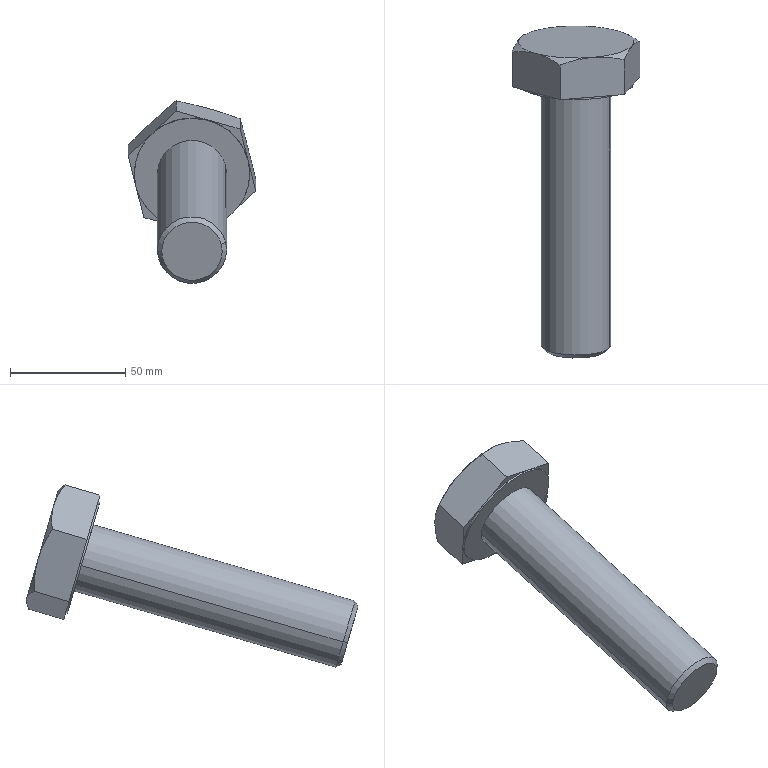Component | SolidWorks | hex structural bolt gradec short_iso-10 | 1 solid | 27 faces | box 55.43 x 143.81 x 78.96 mm | volume 124846 mm3 | plane 15 | cone 8 | cylinder 4 | commonest cylinder face diameters 50 x2 30 x2
STEP:
#1=CARTESIAN_POINT('',(-29.949,-0.9466,13.504));
#2=VERTEX_POINT('',#1);
#3=CARTESIAN_POINT('',(-31.862,-0.8156,13.055));
#4=VERTEX_POINT('',#3);
#5=CARTESIAN_POINT('',(-30.906,-0.8811,13.28));
#6=DIRECTION('',(0.,-0.9601,-0.2797));
#7=DIRECTION('',(0.9713,-0.06652,0.2283));
#8=AXIS2_PLACEMENT_3D('',#5,#6,#7);
#9=CIRCLE('',#8,0.9843);
#10=EDGE_CURVE('',#2,#4,#9,.T.);
#11=ORIENTED_EDGE('',*,*,#10,.F.);
#12=CARTESIAN_POINT('',(-29.949,-0.9163,13.513));
#13=VERTEX_POINT('',#12);
#14=CARTESIAN_POINT('',(-29.949,-0.2397,13.71));
#15=DIRECTION('',(-0.,0.9601,0.2797));
#16=VECTOR('',#15,39.37);
#17=LINE('',#14,#16);
#18=EDGE_CURVE('',#2,#13,#17,.T.);
#19=ORIENTED_EDGE('',*,*,#18,.T.);
#20=CARTESIAN_POINT('',(-30.63,-1.115,14.196));
#21=VERTEX_POINT('',#20);
#22=CARTESIAN_POINT('',(-30.906,-0.8509,13.289));
#23=DIRECTION('',(-0.,0.9601,0.2797));
#24=DIRECTION('',(-0.9713,0.06652,-0.2283));
#25=AXIS2_PLACEMENT_3D('',#22,#23,#24);
#26=CIRCLE('',#25,0.9843);
#27=EDGE_CURVE('',#21,#13,#26,.T.);
#28=ORIENTED_EDGE('',*,*,#27,.F.);
#29=CARTESIAN_POINT('',(-31.586,-1.05,13.971));
#30=VERTEX_POINT('',#29);
#31=CARTESIAN_POINT('',(-30.906,-0.8509,13.289));
#32=DIRECTION('',(-0.,0.9601,0.2797));
#33=DIRECTION('',(-0.9713,0.06652,-0.2283));
#34=AXIS2_PLACEMENT_3D('',#31,#32,#33);
#35=CIRCLE('',#34,0.9843);
#36=EDGE_CURVE('',#30,#21,#35,.T.);
#37=ORIENTED_EDGE('',*,*,#36,.F.);
#38=CARTESIAN_POINT('',(-31.862,-0.7854,13.064));
#39=VERTEX_POINT('',#38);
#40=CARTESIAN_POINT('',(-30.906,-0.8509,13.289));
#41=DIRECTION('',(-0.,0.9601,0.2797));
#42=DIRECTION('',(-0.9713,0.06652,-0.2283));
#43=AXIS2_PLACEMENT_3D('',#40,#41,#42);
#44=CIRCLE('',#43,0.9843);
#45=EDGE_CURVE('',#39,#30,#44,.T.);
#46=ORIENTED_EDGE('',*,*,#45,.F.);
#47=CARTESIAN_POINT('',(-31.862,-0.1088,13.261));
#48=DIRECTION('',(-0.,0.9601,0.2797));
#49=VECTOR('',#48,39.37);
#50=LINE('',#47,#49);
#51=EDGE_CURVE('',#4,#39,#50,.T.);
#52=ORIENTED_EDGE('',*,*,#51,.F.);
#53=EDGE_LOOP('',(#11,#19,#28,#37,#46,#52));
#54=FACE_OUTER_BOUND('',#53,.T.);
#55=CARTESIAN_POINT('',(-30.906,-0.1743,13.486));
#56=DIRECTION('',(-0.,0.9601,0.2797));
#57=DIRECTION('',(-0.9713,0.06652,-0.2283));
#58=AXIS2_PLACEMENT_3D('',#55,#56,#57);
#59=CYLINDRICAL_SURFACE('',#58,0.9843);
#60=ADVANCED_FACE('',(#54),#59,.T.);
#61=CARTESIAN_POINT('',(-31.406,-5.383,11.841));
#62=VERTEX_POINT('',#61);
#63=CARTESIAN_POINT('',(-30.405,-5.451,12.076));
#64=VERTEX_POINT('',#63);
#65=CARTESIAN_POINT('',(-30.906,-5.417,11.958));
#66=DIRECTION('',(-0.,0.9601,0.2797));
#67=DIRECTION('',(-0.9713,0.06652,-0.2283));
#68=AXIS2_PLACEMENT_3D('',#65,#66,#67);
#69=CIRCLE('',#68,0.5149);
#70=EDGE_CURVE('',#62,#64,#69,.T.);
#71=ORIENTED_EDGE('',*,*,#70,.T.);
#72=CARTESIAN_POINT('',(-30.332,-5.384,12.114));
#73=VERTEX_POINT('',#72);
#74=CARTESIAN_POINT('',(-30.405,-5.451,12.076));
#75=DIRECTION('',(0.6868,0.6318,0.3592));
#76=VECTOR('',#75,39.37);
#77=LINE('',#74,#76);
#78=EDGE_CURVE('',#64,#73,#77,.T.);
#79=ORIENTED_EDGE('',*,*,#78,.T.);
#80=CARTESIAN_POINT('',(-31.479,-5.305,11.844));
#81=VERTEX_POINT('',#80);
#82=CARTESIAN_POINT('',(-30.906,-5.344,11.979));
#83=DIRECTION('',(-0.,0.9601,0.2797));
#84=DIRECTION('',(-0.9713,0.06652,-0.2283));
#85=AXIS2_PLACEMENT_3D('',#82,#83,#84);
#86=CIRCLE('',#85,0.5906);
#87=EDGE_CURVE('',#81,#73,#86,.T.);
#88=ORIENTED_EDGE('',*,*,#87,.F.);
#89=CARTESIAN_POINT('',(-31.406,-5.383,11.841));
#90=DIRECTION('',(-0.6868,0.7259,0.03639));
#91=VECTOR('',#90,39.37);
#92=LINE('',#89,#91);
#93=EDGE_CURVE('',#62,#81,#92,.T.);
#94=ORIENTED_EDGE('',*,*,#93,.F.);
#95=EDGE_LOOP('',(#71,#79,#88,#94));
#96=FACE_OUTER_BOUND('',#95,.T.);
#97=CARTESIAN_POINT('',(-30.906,-5.417,11.958));
#98=DIRECTION('',(-0.,0.9601,0.2797));
#99=DIRECTION('',(-0.9713,0.06652,-0.2283));
#100=AXIS2_PLACEMENT_3D('',#97,#98,#99);
#101=CONICAL_SURFACE('',#100,0.5149,0.7854);
#102=ADVANCED_FACE('',(#96),#101,.T.);
#103=ORIENTED_EDGE('',*,*,#87,.T.);
#104=CARTESIAN_POINT('',(-30.332,-0.9204,13.415));
#105=VERTEX_POINT('',#104);
#106=CARTESIAN_POINT('',(-30.332,-0.2135,13.621));
#107=DIRECTION('',(-0.,0.9601,0.2797));
#108=VECTOR('',#107,39.37);
#109=LINE('',#106,#108);
#110=EDGE_CURVE('',#73,#105,#109,.T.);
#111=ORIENTED_EDGE('',*,*,#110,.T.);
#112=CARTESIAN_POINT('',(-31.479,-0.8418,13.145));
#113=VERTEX_POINT('',#112);
#114=CARTESIAN_POINT('',(-30.906,-0.8811,13.28));
#115=DIRECTION('',(-0.,0.9601,0.2797));
#116=DIRECTION('',(0.9713,-0.06652,0.2283));
#117=AXIS2_PLACEMENT_3D('',#114,#115,#116);
#118=CIRCLE('',#117,0.5906);
#119=EDGE_CURVE('',#113,#105,#118,.T.);
#120=ORIENTED_EDGE('',*,*,#119,.F.);
#121=CARTESIAN_POINT('',(-31.479,-0.135,13.351));
#122=DIRECTION('',(-0.,0.9601,0.2797));
#123=VECTOR('',#122,39.37);
#124=LINE('',#121,#123);
#125=EDGE_CURVE('',#81,#113,#124,.T.);
#126=ORIENTED_EDGE('',*,*,#125,.F.);
#127=EDGE_LOOP('',(#103,#111,#120,#126));
#128=FACE_OUTER_BOUND('',#127,.T.);
#129=CARTESIAN_POINT('',(-30.906,-0.1743,13.486));
#130=DIRECTION('',(-0.,0.9601,0.2797));
#131=DIRECTION('',(-0.9713,0.06652,-0.2283));
#132=AXIS2_PLACEMENT_3D('',#129,#130,#131);
#133=CYLINDRICAL_SURFACE('',#132,0.5906);
#134=ADVANCED_FACE('',(#128),#133,.T.);
#135=ORIENTED_EDGE('',*,*,#119,.T.);
#136=CARTESIAN_POINT('',(-30.906,-0.8811,13.28));
#137=DIRECTION('',(-0.,0.9601,0.2797));
#138=DIRECTION('',(0.9713,-0.06652,0.2283));
#139=AXIS2_PLACEMENT_3D('',#136,#137,#138);
#140=CIRCLE('',#139,0.5906);
#141=EDGE_CURVE('',#105,#113,#140,.T.);
#142=ORIENTED_EDGE('',*,*,#141,.T.);
#143=EDGE_LOOP('',(#135,#142));
#144=FACE_BOUND('',#143,.T.);
#145=CARTESIAN_POINT('',(-30.906,-0.8811,13.28));
#146=DIRECTION('',(0.,-0.9601,-0.2797));
#147=DIRECTION('',(0.9713,-0.06652,0.2283));
#148=AXIS2_PLACEMENT_3D('',#145,#146,#147);
#149=CIRCLE('',#148,0.9843);
#150=EDGE_CURVE('',#4,#2,#149,.T.);
#151=ORIENTED_EDGE('',*,*,#150,.T.);
#152=ORIENTED_EDGE('',*,*,#10,.T.);
#153=EDGE_LOOP('',(#151,#152));
#154=FACE_OUTER_BOUND('',#153,.T.);
#155=CARTESIAN_POINT('',(-31.176,-1.19,14.34));
#156=DIRECTION('',(0.,-0.9601,-0.2797));
#157=DIRECTION('',(0.9713,-0.06652,0.2283));
#158=AXIS2_PLACEMENT_3D('',#155,#156,#157);
#159=PLANE('',#158);
#160=ADVANCED_FACE('',(#144,#154),#159,.T.);
#161=ORIENTED_EDGE('',*,*,#110,.F.);
#162=CARTESIAN_POINT('',(-30.906,-5.344,11.979));
#163=DIRECTION('',(-0.,0.9601,0.2797));
#164=DIRECTION('',(-0.9713,0.06652,-0.2283));
#165=AXIS2_PLACEMENT_3D('',#162,#163,#164);
#166=CIRCLE('',#165,0.5906);
#167=EDGE_CURVE('',#73,#81,#166,.T.);
#168=ORIENTED_EDGE('',*,*,#167,.T.);
#169=ORIENTED_EDGE('',*,*,#125,.T.);
#170=ORIENTED_EDGE('',*,*,#141,.F.);
#171=EDGE_LOOP('',(#161,#168,#169,#170));
#172=FACE_OUTER_BOUND('',#171,.T.);
#173=CARTESIAN_POINT('',(-30.906,-0.1743,13.486));
#174=DIRECTION('',(-0.,0.9601,0.2797));
#175=DIRECTION('',(-0.9713,0.06652,-0.2283));
#176=AXIS2_PLACEMENT_3D('',#173,#174,#175);
#177=CYLINDRICAL_SURFACE('',#176,0.5906);
#178=ADVANCED_FACE('',(#172),#177,.T.);
#179=ORIENTED_EDGE('',*,*,#78,.F.);
#180=CARTESIAN_POINT('',(-30.906,-5.417,11.958));
#181=DIRECTION('',(-0.,0.9601,0.2797));
#182=DIRECTION('',(-0.9713,0.06652,-0.2283));
#183=AXIS2_PLACEMENT_3D('',#180,#181,#182);
#184=CIRCLE('',#183,0.5149);
#185=EDGE_CURVE('',#64,#62,#184,.T.);
#186=ORIENTED_EDGE('',*,*,#185,.T.);
#187=ORIENTED_EDGE('',*,*,#93,.T.);
#188=ORIENTED_EDGE('',*,*,#167,.F.);
#189=EDGE_LOOP('',(#179,#186,#187,#188));
#190=FACE_OUTER_BOUND('',#189,.T.);
#191=CARTESIAN_POINT('',(-30.906,-5.417,11.958));
#192=DIRECTION('',(-0.,0.9601,0.2797));
#193=DIRECTION('',(-0.9713,0.06652,-0.2283));
#194=AXIS2_PLACEMENT_3D('',#191,#192,#193);
#195=CONICAL_SURFACE('',#194,0.5149,0.7854);
#196=ADVANCED_FACE('',(#190),#195,.T.);
#197=ORIENTED_EDGE('',*,*,#70,.F.);
#198=ORIENTED_EDGE('',*,*,#185,.F.);
#199=EDGE_LOOP('',(#197,#198));
#200=FACE_OUTER_BOUND('',#199,.T.);
#201=CARTESIAN_POINT('',(-30.906,-5.417,11.958));
#202=DIRECTION('',(-0.,0.9601,0.2797));
#203=DIRECTION('',(-0.9713,0.06652,-0.2283));
#204=AXIS2_PLACEMENT_3D('',#201,#202,#203);
#205=PLANE('',#204);
#206=ADVANCED_FACE('',(#200),#205,.F.);
#207=CARTESIAN_POINT('',(-30.085,-1.071,14.043));
#208=VERTEX_POINT('',#207);
#209=CARTESIAN_POINT('',(-30.085,-1.071,14.043));
#210=DIRECTION('',(-0.9601,-0.07826,0.2686));
#211=VECTOR('',#210,39.37);
#212=LINE('',#209,#211);
#213=EDGE_CURVE('',#208,#21,#212,.T.);
#214=ORIENTED_EDGE('',*,*,#213,.T.);
#215=ORIENTED_EDGE('',*,*,#27,.T.);
#216=CARTESIAN_POINT('',(-30.085,-1.071,14.043));
#217=DIRECTION('',(-0.2378,-0.2717,0.9325));
#218=VECTOR('',#217,39.37);
#219=LINE('',#216,#218);
#220=EDGE_CURVE('',#13,#208,#219,.T.);
#221=ORIENTED_EDGE('',*,*,#220,.T.);
#222=EDGE_LOOP('',(#214,#215,#221));
#223=FACE_OUTER_BOUND('',#222,.T.);
#224=CARTESIAN_POINT('',(-31.14,-1.118,14.206));
#225=DIRECTION('',(0.,-0.9601,-0.2797));
#226=DIRECTION('',(0.9713,-0.06652,0.2283));
#227=AXIS2_PLACEMENT_3D('',#224,#225,#226);
#228=PLANE('',#227);
#229=ADVANCED_FACE('',(#223),#228,.T.);
#230=CARTESIAN_POINT('',(-31.176,-1.16,14.348));
#231=VERTEX_POINT('',#230);
#232=CARTESIAN_POINT('',(-30.085,-1.071,14.043));
#233=DIRECTION('',(-0.9601,-0.07826,0.2686));
#234=VECTOR('',#233,39.37);
#235=LINE('',#232,#234);
#236=EDGE_CURVE('',#21,#231,#235,.T.);
#237=ORIENTED_EDGE('',*,*,#236,.T.);
#238=CARTESIAN_POINT('',(-31.176,-1.16,14.348));
#239=DIRECTION('',(-0.7223,0.1935,-0.664));
#240=VECTOR('',#239,39.37);
#241=LINE('',#238,#240);
#242=EDGE_CURVE('',#231,#30,#241,.T.);
#243=ORIENTED_EDGE('',*,*,#242,.T.);
#244=ORIENTED_EDGE('',*,*,#36,.T.);
#245=EDGE_LOOP('',(#237,#243,#244));
#246=FACE_OUTER_BOUND('',#245,.T.);
#247=CARTESIAN_POINT('',(-31.14,-1.118,14.206));
#248=DIRECTION('',(0.,-0.9601,-0.2797));
#249=DIRECTION('',(0.9713,-0.06652,0.2283));
#250=AXIS2_PLACEMENT_3D('',#247,#248,#249);
#251=PLANE('',#250);
#252=ADVANCED_FACE('',(#246),#251,.T.);
#253=CARTESIAN_POINT('',(-31.997,-0.9398,13.594));
#254=VERTEX_POINT('',#253);
#255=CARTESIAN_POINT('',(-31.176,-1.16,14.348));
#256=DIRECTION('',(-0.7223,0.1935,-0.664));
#257=VECTOR('',#256,39.37);
#258=LINE('',#255,#257);
#259=EDGE_CURVE('',#30,#254,#258,.T.);
#260=ORIENTED_EDGE('',*,*,#259,.T.);
#261=CARTESIAN_POINT('',(-31.997,-0.9398,13.594));
#262=DIRECTION('',(0.2378,0.2717,-0.9325));
#263=VECTOR('',#262,39.37);
#264=LINE('',#261,#263);
#265=EDGE_CURVE('',#254,#39,#264,.T.);
#266=ORIENTED_EDGE('',*,*,#265,.T.);
#267=ORIENTED_EDGE('',*,*,#45,.T.);
#268=EDGE_LOOP('',(#260,#266,#267));
#269=FACE_OUTER_BOUND('',#268,.T.);
#270=CARTESIAN_POINT('',(-31.14,-1.118,14.206));
#271=DIRECTION('',(0.,-0.9601,-0.2797));
#272=DIRECTION('',(0.9713,-0.06652,0.2283));
#273=AXIS2_PLACEMENT_3D('',#270,#271,#272);
#274=PLANE('',#273);
#275=ADVANCED_FACE('',(#269),#274,.T.);
#276=CARTESIAN_POINT('',(-31.726,-0.631,12.534));
#277=VERTEX_POINT('',#276);
#278=CARTESIAN_POINT('',(-31.997,-0.9398,13.594));
#279=DIRECTION('',(0.2378,0.2717,-0.9325));
#280=VECTOR('',#279,39.37);
#281=LINE('',#278,#280);
#282=EDGE_CURVE('',#39,#277,#281,.T.);
#283=ORIENTED_EDGE('',*,*,#282,.T.);
#284=CARTESIAN_POINT('',(-31.181,-0.5865,12.381));
#285=VERTEX_POINT('',#284);
#286=CARTESIAN_POINT('',(-30.635,-0.542,12.229));
#287=DIRECTION('',(0.9601,0.07826,-0.2686));
#288=VECTOR('',#287,39.37);
#289=LINE('',#286,#288);
#290=EDGE_CURVE('',#277,#285,#289,.T.);
#291=ORIENTED_EDGE('',*,*,#290,.T.);
#292=CARTESIAN_POINT('',(-30.906,-0.8509,13.289));
#293=DIRECTION('',(-0.,0.9601,0.2797));
#294=DIRECTION('',(-0.9713,0.06652,-0.2283));
#295=AXIS2_PLACEMENT_3D('',#292,#293,#294);
#296=CIRCLE('',#295,0.9843);
#297=EDGE_CURVE('',#285,#39,#296,.T.);
#298=ORIENTED_EDGE('',*,*,#297,.T.);
#299=EDGE_LOOP('',(#283,#291,#298));
#300=FACE_OUTER_BOUND('',#299,.T.);
#301=CARTESIAN_POINT('',(-31.14,-1.118,14.206));
#302=DIRECTION('',(0.,-0.9601,-0.2797));
#303=DIRECTION('',(0.9713,-0.06652,0.2283));
#304=AXIS2_PLACEMENT_3D('',#301,#302,#303);
#305=PLANE('',#304);
#306=ADVANCED_FACE('',(#300),#305,.T.);
#307=CARTESIAN_POINT('',(-30.635,-0.542,12.229));
#308=VERTEX_POINT('',#307);
#309=CARTESIAN_POINT('',(-30.635,-0.542,12.229));
#310=DIRECTION('',(0.9601,0.07826,-0.2686));
#311=VECTOR('',#310,39.37);
#312=LINE('',#309,#311);
#313=EDGE_CURVE('',#285,#308,#312,.T.);
#314=ORIENTED_EDGE('',*,*,#313,.T.);
#315=CARTESIAN_POINT('',(-30.225,-0.652,12.606));
#316=VERTEX_POINT('',#315);
#317=CARTESIAN_POINT('',(-29.814,-0.7619,12.983));
#318=DIRECTION('',(0.7223,-0.1935,0.664));
#319=VECTOR('',#318,39.37);
#320=LINE('',#317,#319);
#321=EDGE_CURVE('',#308,#316,#320,.T.);
#322=ORIENTED_EDGE('',*,*,#321,.T.);
#323=CARTESIAN_POINT('',(-30.906,-0.8509,13.289));
#324=DIRECTION('',(-0.,0.9601,0.2797));
#325=DIRECTION('',(-0.9713,0.06652,-0.2283));
#326=AXIS2_PLACEMENT_3D('',#323,#324,#325);
#327=CIRCLE('',#326,0.9843);
#328=EDGE_CURVE('',#316,#285,#327,.T.);
#329=ORIENTED_EDGE('',*,*,#328,.T.);
#330=EDGE_LOOP('',(#314,#322,#329));
#331=FACE_OUTER_BOUND('',#330,.T.);
#332=CARTESIAN_POINT('',(-31.14,-1.118,14.206));
#333=DIRECTION('',(0.,-0.9601,-0.2797));
#334=DIRECTION('',(0.9713,-0.06652,0.2283));
#335=AXIS2_PLACEMENT_3D('',#332,#333,#334);
#336=PLANE('',#335);
#337=ADVANCED_FACE('',(#331),#336,.T.);
#338=CARTESIAN_POINT('',(-29.814,-0.7619,12.983));
#339=VERTEX_POINT('',#338);
#340=CARTESIAN_POINT('',(-29.814,-0.7619,12.983));
#341=DIRECTION('',(0.7223,-0.1935,0.664));
#342=VECTOR('',#341,39.37);
#343=LINE('',#340,#342);
#344=EDGE_CURVE('',#316,#339,#343,.T.);
#345=ORIENTED_EDGE('',*,*,#344,.T.);
#346=CARTESIAN_POINT('',(-30.085,-1.071,14.043));
#347=DIRECTION('',(-0.2378,-0.2717,0.9325));
#348=VECTOR('',#347,39.37);
#349=LINE('',#346,#348);
#350=EDGE_CURVE('',#339,#13,#349,.T.);
#351=ORIENTED_EDGE('',*,*,#350,.T.);
#352=CARTESIAN_POINT('',(-30.906,-0.8509,13.289));
#353=DIRECTION('',(-0.,0.9601,0.2797));
#354=DIRECTION('',(-0.9713,0.06652,-0.2283));
#355=AXIS2_PLACEMENT_3D('',#352,#353,#354);
#356=CIRCLE('',#355,0.9843);
#357=EDGE_CURVE('',#13,#316,#356,.T.);
#358=ORIENTED_EDGE('',*,*,#357,.T.);
#359=EDGE_LOOP('',(#345,#351,#358));
#360=FACE_OUTER_BOUND('',#359,.T.);
#361=CARTESIAN_POINT('',(-31.14,-1.118,14.206));
#362=DIRECTION('',(0.,-0.9601,-0.2797));
#363=DIRECTION('',(0.9713,-0.06652,0.2283));
#364=AXIS2_PLACEMENT_3D('',#361,#362,#363);
#365=PLANE('',#364);
#366=ADVANCED_FACE('',(#360),#365,.T.);
#367=ORIENTED_EDGE('',*,*,#18,.F.);
#368=ORIENTED_EDGE('',*,*,#150,.F.);
#369=ORIENTED_EDGE('',*,*,#51,.T.);
#370=ORIENTED_EDGE('',*,*,#297,.F.);
#371=ORIENTED_EDGE('',*,*,#328,.F.);
#372=ORIENTED_EDGE('',*,*,#357,.F.);
#373=EDGE_LOOP('',(#367,#368,#369,#370,#371,#372));
#374=FACE_OUTER_BOUND('',#373,.T.);
#375=CARTESIAN_POINT('',(-30.906,-0.1743,13.486));
#376=DIRECTION('',(-0.,0.9601,0.2797));
#377=DIRECTION('',(-0.9713,0.06652,-0.2283));
#378=AXIS2_PLACEMENT_3D('',#375,#376,#377);
#379=CYLINDRICAL_SURFACE('',#378,0.9843);
#380=ADVANCED_FACE('',(#374),#379,.T.);
#381=CARTESIAN_POINT('',(-29.949,-0.2397,13.71));
#382=VERTEX_POINT('',#381);
#383=CARTESIAN_POINT('',(-30.63,-0.4386,14.393));
#384=VERTEX_POINT('',#383);
#385=CARTESIAN_POINT('',(-30.906,-0.1743,13.486));
#386=DIRECTION('',(0.,-0.9601,-0.2797));
#387=DIRECTION('',(0.9713,-0.06652,0.2283));
#388=AXIS2_PLACEMENT_3D('',#385,#386,#387);
#389=CIRCLE('',#388,0.9843);
#390=EDGE_CURVE('',#382,#384,#389,.T.);
#391=ORIENTED_EDGE('',*,*,#390,.F.);
#392=CARTESIAN_POINT('',(-30.225,0.02462,12.803));
#393=VERTEX_POINT('',#392);
#394=CARTESIAN_POINT('',(-30.906,-0.1743,13.486));
#395=DIRECTION('',(0.,-0.9601,-0.2797));
#396=DIRECTION('',(0.9713,-0.06652,0.2283));
#397=AXIS2_PLACEMENT_3D('',#394,#395,#396);
#398=CIRCLE('',#397,0.9843);
#399=EDGE_CURVE('',#393,#382,#398,.T.);
#400=ORIENTED_EDGE('',*,*,#399,.F.);
#401=CARTESIAN_POINT('',(-31.181,0.09008,12.578));
#402=VERTEX_POINT('',#401);
#403=CARTESIAN_POINT('',(-30.906,-0.1743,13.486));
#404=DIRECTION('',(0.,-0.9601,-0.2797));
#405=DIRECTION('',(0.9713,-0.06652,0.2283));
#406=AXIS2_PLACEMENT_3D('',#403,#404,#405);
#407=CIRCLE('',#406,0.9843);
#408=EDGE_CURVE('',#402,#393,#407,.T.);
#409=ORIENTED_EDGE('',*,*,#408,.F.);
#410=CARTESIAN_POINT('',(-31.862,-0.1088,13.261));
#411=VERTEX_POINT('',#410);
#412=CARTESIAN_POINT('',(-30.906,-0.1743,13.486));
#413=DIRECTION('',(0.,-0.9601,-0.2797));
#414=DIRECTION('',(0.9713,-0.06652,0.2283));
#415=AXIS2_PLACEMENT_3D('',#412,#413,#414);
#416=CIRCLE('',#415,0.9843);
#417=EDGE_CURVE('',#411,#402,#416,.T.);
#418=ORIENTED_EDGE('',*,*,#417,.F.);
#419=CARTESIAN_POINT('',(-31.586,-0.3731,14.168));
#420=VERTEX_POINT('',#419);
#421=CARTESIAN_POINT('',(-30.906,-0.1743,13.486));
#422=DIRECTION('',(-0.,0.9601,0.2797));
#423=DIRECTION('',(-0.9713,0.06652,-0.2283));
#424=AXIS2_PLACEMENT_3D('',#421,#422,#423);
#425=CIRCLE('',#424,0.9843);
#426=EDGE_CURVE('',#411,#420,#425,.T.);
#427=ORIENTED_EDGE('',*,*,#426,.T.);
#428=CARTESIAN_POINT('',(-30.906,-0.1743,13.486));
#429=DIRECTION('',(0.,-0.9601,-0.2797));
#430=DIRECTION('',(0.9713,-0.06652,0.2283));
#431=AXIS2_PLACEMENT_3D('',#428,#429,#430);
#432=CIRCLE('',#431,0.9843);
#433=EDGE_CURVE('',#384,#420,#432,.T.);
#434=ORIENTED_EDGE('',*,*,#433,.F.);
#435=EDGE_LOOP('',(#391,#400,#409,#418,#427,#434));
#436=FACE_OUTER_BOUND('',#435,.T.);
#437=CARTESIAN_POINT('',(-31.176,-0.4831,14.546));
#438=DIRECTION('',(0.,-0.9601,-0.2797));
#439=DIRECTION('',(0.9713,-0.06652,0.2283));
#440=AXIS2_PLACEMENT_3D('',#437,#438,#439);
#441=PLANE('',#440);
#442=ADVANCED_FACE('',(#436),#441,.F.);
#443=CARTESIAN_POINT('',(-31.176,-0.5675,14.521));
#444=VERTEX_POINT('',#443);
#445=CARTESIAN_POINT('',(-31.586,-0.3731,14.168));
#446=CARTESIAN_POINT('',(-31.569,-0.3778,14.184));
#447=CARTESIAN_POINT('',(-31.551,-0.383,14.2));
#448=CARTESIAN_POINT('',(-31.516,-0.3943,14.232));
#449=CARTESIAN_POINT('',(-31.499,-0.4004,14.247));
#450=CARTESIAN_POINT('',(-31.447,-0.4201,14.293));
#451=CARTESIAN_POINT('',(-31.413,-0.435,14.323));
#452=CARTESIAN_POINT('',(-31.31,-0.4845,14.411));
#453=CARTESIAN_POINT('',(-31.243,-0.5238,14.467));
#454=CARTESIAN_POINT('',(-31.176,-0.5675,14.521));
#455=B_SPLINE_CURVE_WITH_KNOTS('',3,(#445,#446,#447,#448,#449,#450,#451,#452,#453,#454),.UNSPECIFIED.,.F.,.F.,(4,2,2,2,4),(0.0146,0.01642,0.01824,0.02188,0.02915),.UNSPECIFIED.);
#456=EDGE_CURVE('',#420,#444,#455,.T.);
#457=ORIENTED_EDGE('',*,*,#456,.T.);
#458=CARTESIAN_POINT('',(-31.176,-0.5675,14.521));
#459=CARTESIAN_POINT('',(-31.086,-0.5344,14.504));
#460=CARTESIAN_POINT('',(-30.997,-0.5059,14.485));
#461=CARTESIAN_POINT('',(-30.815,-0.4617,14.442));
#462=CARTESIAN_POINT('',(-30.723,-0.4462,14.419));
#463=CARTESIAN_POINT('',(-30.63,-0.4386,14.393));
#464=B_SPLINE_CURVE_WITH_KNOTS('',3,(#458,#459,#460,#461,#462,#463),.UNSPECIFIED.,.F.,.F.,(4,2,4),(0.00000024,0.007303,0.0146),.UNSPECIFIED.);
#465=EDGE_CURVE('',#444,#384,#464,.T.);
#466=ORIENTED_EDGE('',*,*,#465,.T.);
#467=ORIENTED_EDGE('',*,*,#433,.T.);
#468=EDGE_LOOP('',(#457,#466,#467));
#469=FACE_OUTER_BOUND('',#468,.T.);
#470=CARTESIAN_POINT('',(-30.906,-0.1743,13.486));
#471=DIRECTION('',(0.,-0.9601,-0.2797));
#472=DIRECTION('',(0.9713,-0.06652,0.2283));
#473=AXIS2_PLACEMENT_3D('',#470,#471,#472);
#474=CONICAL_SURFACE('',#473,0.9843,1.047);
#475=ADVANCED_FACE('',(#469),#474,.T.);
#476=CARTESIAN_POINT('',(-31.997,-0.3476,13.766));
#477=VERTEX_POINT('',#476);
#478=CARTESIAN_POINT('',(-31.862,-0.1088,13.261));
#479=CARTESIAN_POINT('',(-31.873,-0.1219,13.306));
#480=CARTESIAN_POINT('',(-31.884,-0.1369,13.35));
#481=CARTESIAN_POINT('',(-31.907,-0.171,13.438));
#482=CARTESIAN_POINT('',(-31.919,-0.1898,13.481));
#483=CARTESIAN_POINT('',(-31.953,-0.2507,13.607));
#484=CARTESIAN_POINT('',(-31.975,-0.2972,13.688));
#485=CARTESIAN_POINT('',(-31.997,-0.3476,13.766));
#486=B_SPLINE_CURVE_WITH_KNOTS('',3,(#478,#479,#480,#481,#482,#483,#484,#485),.UNSPECIFIED.,.F.,.F.,(4,2,2,4),(0.0408,0.04446,0.04811,0.05542),.UNSPECIFIED.);
#487=EDGE_CURVE('',#411,#477,#486,.T.);
#488=ORIENTED_EDGE('',*,*,#487,.T.);
#489=CARTESIAN_POINT('',(-31.997,-0.3476,13.766));
#490=CARTESIAN_POINT('',(-31.93,-0.3398,13.836));
#491=CARTESIAN_POINT('',(-31.862,-0.3367,13.904));
#492=CARTESIAN_POINT('',(-31.725,-0.344,14.038));
#493=CARTESIAN_POINT('',(-31.656,-0.3544,14.104));
#494=CARTESIAN_POINT('',(-31.586,-0.3731,14.168));
#495=B_SPLINE_CURVE_WITH_KNOTS('',3,(#489,#490,#491,#492,#493,#494),.UNSPECIFIED.,.F.,.F.,(4,2,4),(0.00000024,0.007303,0.0146),.UNSPECIFIED.);
#496=EDGE_CURVE('',#477,#420,#495,.T.);
#497=ORIENTED_EDGE('',*,*,#496,.T.);
#498=ORIENTED_EDGE('',*,*,#426,.F.);
#499=EDGE_LOOP('',(#488,#497,#498));
#500=FACE_OUTER_BOUND('',#499,.T.);
#501=CARTESIAN_POINT('',(-30.906,-0.1743,13.486));
#502=DIRECTION('',(0.,-0.9601,-0.2797));
#503=DIRECTION('',(0.9713,-0.06652,0.2283));
#504=AXIS2_PLACEMENT_3D('',#501,#502,#503);
#505=CONICAL_SURFACE('',#504,0.9843,1.047);
#506=ADVANCED_FACE('',(#500),#505,.T.);
#507=CARTESIAN_POINT('',(-31.726,-0.03879,12.707));
#508=VERTEX_POINT('',#507);
#509=CARTESIAN_POINT('',(-31.726,-0.03879,12.707));
#510=CARTESIAN_POINT('',(-31.737,-0.03854,12.753));
#511=CARTESIAN_POINT('',(-31.749,-0.03945,12.8));
#512=CARTESIAN_POINT('',(-31.771,-0.04423,12.894));
#513=CARTESIAN_POINT('',(-31.782,-0.04807,12.941));
#514=CARTESIAN_POINT('',(-31.816,-0.0647,13.08));
#515=CARTESIAN_POINT('',(-31.839,-0.08269,13.171));
#516=CARTESIAN_POINT('',(-31.862,-0.1088,13.261));
#517=B_SPLINE_CURVE_WITH_KNOTS('',3,(#509,#510,#511,#512,#513,#514,#515,#516),.UNSPECIFIED.,.F.,.F.,(4,2,2,4),(0.0262,0.02985,0.0335,0.0408),.UNSPECIFIED.);
#518=EDGE_CURVE('',#508,#411,#517,.T.);
#519=ORIENTED_EDGE('',*,*,#518,.T.);
#520=ORIENTED_EDGE('',*,*,#417,.T.);
#521=CARTESIAN_POINT('',(-31.181,0.09008,12.578));
#522=CARTESIAN_POINT('',(-31.204,0.0882,12.585));
#523=CARTESIAN_POINT('',(-31.227,0.0858,12.591));
#524=CARTESIAN_POINT('',(-31.274,0.08007,12.604));
#525=CARTESIAN_POINT('',(-31.297,0.07672,12.61));
#526=CARTESIAN_POINT('',(-31.366,0.0653,12.627));
#527=CARTESIAN_POINT('',(-31.411,0.05586,12.638));
#528=CARTESIAN_POINT('',(-31.548,0.0227,12.67));
#529=CARTESIAN_POINT('',(-31.637,-0.005831,12.689));
#530=CARTESIAN_POINT('',(-31.726,-0.03879,12.707));
#531=B_SPLINE_CURVE_WITH_KNOTS('',3,(#521,#522,#523,#524,#525,#526,#527,#528,#529,#530),.UNSPECIFIED.,.F.,.F.,(4,2,2,2,4),(0.0146,0.01642,0.01824,0.02188,0.02915),.UNSPECIFIED.);
#532=EDGE_CURVE('',#402,#508,#531,.T.);
#533=ORIENTED_EDGE('',*,*,#532,.T.);
#534=EDGE_LOOP('',(#519,#520,#533));
#535=FACE_OUTER_BOUND('',#534,.T.);
#536=CARTESIAN_POINT('',(-30.906,-0.1743,13.486));
#537=DIRECTION('',(0.,-0.9601,-0.2797));
#538=DIRECTION('',(0.9713,-0.06652,0.2283));
#539=AXIS2_PLACEMENT_3D('',#536,#537,#538);
#540=CONICAL_SURFACE('',#539,0.9843,1.047);
#541=ADVANCED_FACE('',(#535),#540,.T.);
#542=CARTESIAN_POINT('',(-30.635,0.05015,12.401));
#543=VERTEX_POINT('',#542);
#544=CARTESIAN_POINT('',(-30.635,0.05015,12.401));
#545=CARTESIAN_POINT('',(-30.725,0.06864,12.434));
#546=CARTESIAN_POINT('',(-30.814,0.08254,12.465));
#547=CARTESIAN_POINT('',(-30.996,0.0971,12.524));
#548=CARTESIAN_POINT('',(-31.088,0.09766,12.552));
#549=CARTESIAN_POINT('',(-31.181,0.09008,12.578));
#550=B_SPLINE_CURVE_WITH_KNOTS('',3,(#544,#545,#546,#547,#548,#549),.UNSPECIFIED.,.F.,.F.,(4,2,4),(0.00000024,0.007303,0.0146),.UNSPECIFIED.);
#551=EDGE_CURVE('',#543,#402,#550,.T.);
#552=ORIENTED_EDGE('',*,*,#551,.T.);
#553=ORIENTED_EDGE('',*,*,#408,.T.);
#554=CARTESIAN_POINT('',(-30.225,0.02462,12.803));
#555=CARTESIAN_POINT('',(-30.242,0.02928,12.787));
#556=CARTESIAN_POINT('',(-30.26,0.03347,12.771));
#557=CARTESIAN_POINT('',(-30.295,0.04084,12.738));
#558=CARTESIAN_POINT('',(-30.312,0.04403,12.722));
#559=CARTESIAN_POINT('',(-30.364,0.05214,12.673));
#560=CARTESIAN_POINT('',(-30.398,0.05563,12.639));
#561=CARTESIAN_POINT('',(-30.501,0.06104,12.539));
#562=CARTESIAN_POINT('',(-30.568,0.05791,12.47));
#563=CARTESIAN_POINT('',(-30.635,0.05015,12.401));
#564=B_SPLINE_CURVE_WITH_KNOTS('',3,(#554,#555,#556,#557,#558,#559,#560,#561,#562,#563),.UNSPECIFIED.,.F.,.F.,(4,2,2,2,4),(0.0146,0.01642,0.01824,0.02188,0.02915),.UNSPECIFIED.);
#565=EDGE_CURVE('',#393,#543,#564,.T.);
#566=ORIENTED_EDGE('',*,*,#565,.T.);
#567=EDGE_LOOP('',(#552,#553,#566));
#568=FACE_OUTER_BOUND('',#567,.T.);
#569=CARTESIAN_POINT('',(-30.906,-0.1743,13.486));
#570=DIRECTION('',(0.,-0.9601,-0.2797));
#571=DIRECTION('',(0.9713,-0.06652,0.2283));
#572=AXIS2_PLACEMENT_3D('',#569,#570,#571);
#573=CONICAL_SURFACE('',#572,0.9843,1.047);
#574=ADVANCED_FACE('',(#568),#573,.T.);
#575=CARTESIAN_POINT('',(-30.085,-0.4785,14.216));
#576=VERTEX_POINT('',#575);
#577=CARTESIAN_POINT('',(-30.63,-0.4386,14.393));
#578=CARTESIAN_POINT('',(-30.607,-0.4367,14.386));
#579=CARTESIAN_POINT('',(-30.584,-0.4353,14.38));
#580=CARTESIAN_POINT('',(-30.537,-0.4335,14.366));
#581=CARTESIAN_POINT('',(-30.514,-0.4331,14.359));
#582=CARTESIAN_POINT('',(-30.445,-0.4333,14.338));
#583=CARTESIAN_POINT('',(-30.4,-0.4353,14.324));
#584=CARTESIAN_POINT('',(-30.263,-0.4462,14.279));
#585=CARTESIAN_POINT('',(-30.174,-0.4601,14.248));
#586=CARTESIAN_POINT('',(-30.085,-0.4785,14.216));
#587=B_SPLINE_CURVE_WITH_KNOTS('',3,(#577,#578,#579,#580,#581,#582,#583,#584,#585,#586),.UNSPECIFIED.,.F.,.F.,(4,2,2,2,4),(0.0146,0.01642,0.01824,0.02188,0.02915),.UNSPECIFIED.);
#588=EDGE_CURVE('',#384,#576,#587,.T.);
#589=ORIENTED_EDGE('',*,*,#588,.T.);
#590=CARTESIAN_POINT('',(-30.085,-0.4785,14.216));
#591=CARTESIAN_POINT('',(-30.063,-0.4281,14.137));
#592=CARTESIAN_POINT('',(-30.041,-0.3816,14.057));
#593=CARTESIAN_POINT('',(-30.007,-0.3208,13.931));
#594=CARTESIAN_POINT('',(-29.995,-0.302,13.888));
#595=CARTESIAN_POINT('',(-29.972,-0.2679,13.8));
#596=CARTESIAN_POINT('',(-29.961,-0.2528,13.755));
#597=CARTESIAN_POINT('',(-29.949,-0.2397,13.71));
#598=B_SPLINE_CURVE_WITH_KNOTS('',3,(#590,#591,#592,#593,#594,#595,#596,#597),.UNSPECIFIED.,.F.,.F.,(4,2,2,4),(0.06452,0.07184,0.07549,0.07915),.UNSPECIFIED.);
#599=EDGE_CURVE('',#576,#382,#598,.T.);
#600=ORIENTED_EDGE('',*,*,#599,.T.);
#601=ORIENTED_EDGE('',*,*,#390,.T.);
#602=EDGE_LOOP('',(#589,#600,#601));
#603=FACE_OUTER_BOUND('',#602,.T.);
#604=CARTESIAN_POINT('',(-30.906,-0.1743,13.486));
#605=DIRECTION('',(0.,-0.9601,-0.2797));
#606=DIRECTION('',(0.9713,-0.06652,0.2283));
#607=AXIS2_PLACEMENT_3D('',#604,#605,#606);
#608=CONICAL_SURFACE('',#607,0.9843,1.047);
#609=ADVANCED_FACE('',(#603),#608,.T.);
#610=CARTESIAN_POINT('',(-29.814,-0.1697,13.156));
#611=VERTEX_POINT('',#610);
#612=CARTESIAN_POINT('',(-29.814,-0.1697,13.156));
#613=CARTESIAN_POINT('',(-29.882,-0.126,13.102));
#614=CARTESIAN_POINT('',(-29.949,-0.08663,13.046));
#615=CARTESIAN_POINT('',(-30.086,-0.02066,12.929));
#616=CARTESIAN_POINT('',(-30.155,0.005886,12.867));
#617=CARTESIAN_POINT('',(-30.225,0.02462,12.803));
#618=B_SPLINE_CURVE_WITH_KNOTS('',3,(#612,#613,#614,#615,#616,#617),.UNSPECIFIED.,.F.,.F.,(4,2,4),(0.00000024,0.007303,0.0146),.UNSPECIFIED.);
#619=EDGE_CURVE('',#611,#393,#618,.T.);
#620=ORIENTED_EDGE('',*,*,#619,.T.);
#621=ORIENTED_EDGE('',*,*,#399,.T.);
#622=CARTESIAN_POINT('',(-29.949,-0.2397,13.71));
#623=CARTESIAN_POINT('',(-29.927,-0.2136,13.621));
#624=CARTESIAN_POINT('',(-29.904,-0.1956,13.53));
#625=CARTESIAN_POINT('',(-29.87,-0.179,13.39));
#626=CARTESIAN_POINT('',(-29.859,-0.1752,13.344));
#627=CARTESIAN_POINT('',(-29.836,-0.1704,13.25));
#628=CARTESIAN_POINT('',(-29.825,-0.1695,13.203));
#629=CARTESIAN_POINT('',(-29.814,-0.1697,13.156));
#630=B_SPLINE_CURVE_WITH_KNOTS('',3,(#622,#623,#624,#625,#626,#627,#628,#629),.UNSPECIFIED.,.F.,.F.,(4,2,2,4),(0.07915,0.08646,0.09011,0.09377),.UNSPECIFIED.);
#631=EDGE_CURVE('',#382,#611,#630,.T.);
#632=ORIENTED_EDGE('',*,*,#631,.T.);
#633=EDGE_LOOP('',(#620,#621,#632));
#634=FACE_OUTER_BOUND('',#633,.T.);
#635=CARTESIAN_POINT('',(-30.906,-0.1743,13.486));
#636=DIRECTION('',(0.,-0.9601,-0.2797));
#637=DIRECTION('',(0.9713,-0.06652,0.2283));
#638=AXIS2_PLACEMENT_3D('',#635,#636,#637);
#639=CONICAL_SURFACE('',#638,0.9843,1.047);
#640=ADVANCED_FACE('',(#634),#639,.T.);
#641=ORIENTED_EDGE('',*,*,#350,.F.);
#642=CARTESIAN_POINT('',(-29.814,-0.7921,12.975));
#643=DIRECTION('',(-0.,0.9601,0.2797));
#644=VECTOR('',#643,39.37);
#645=LINE('',#642,#644);
#646=EDGE_CURVE('',#339,#611,#645,.T.);
#647=ORIENTED_EDGE('',*,*,#646,.T.);
#648=ORIENTED_EDGE('',*,*,#631,.F.);
#649=ORIENTED_EDGE('',*,*,#599,.F.);
#650=CARTESIAN_POINT('',(-30.085,-1.101,14.034));
#651=DIRECTION('',(-0.,0.9601,0.2797));
#652=VECTOR('',#651,39.37);
#653=LINE('',#650,#652);
#654=EDGE_CURVE('',#208,#576,#653,.T.);
#655=ORIENTED_EDGE('',*,*,#654,.F.);
#656=ORIENTED_EDGE('',*,*,#220,.F.);
#657=EDGE_LOOP('',(#641,#647,#648,#649,#655,#656));
#658=FACE_OUTER_BOUND('',#657,.T.);
#659=CARTESIAN_POINT('',(-30.085,-1.101,14.034));
#660=DIRECTION('',(-0.9713,0.06652,-0.2283));
#661=DIRECTION('',(0.2378,0.2717,-0.9325));
#662=AXIS2_PLACEMENT_3D('',#659,#660,#661);
#663=PLANE('',#662);
#664=ADVANCED_FACE('',(#658),#663,.F.);
#665=ORIENTED_EDGE('',*,*,#321,.F.);
#666=CARTESIAN_POINT('',(-30.635,-0.5723,12.22));
#667=DIRECTION('',(-0.,0.9601,0.2797));
#668=VECTOR('',#667,39.37);
#669=LINE('',#666,#668);
#670=EDGE_CURVE('',#308,#543,#669,.T.);
#671=ORIENTED_EDGE('',*,*,#670,.T.);
#672=ORIENTED_EDGE('',*,*,#565,.F.);
#673=ORIENTED_EDGE('',*,*,#619,.F.);
#674=ORIENTED_EDGE('',*,*,#646,.F.);
#675=ORIENTED_EDGE('',*,*,#344,.F.);
#676=EDGE_LOOP('',(#665,#671,#672,#673,#674,#675));
#677=FACE_OUTER_BOUND('',#676,.T.);
#678=CARTESIAN_POINT('',(-29.814,-0.7921,12.975));
#679=DIRECTION('',(-0.6916,-0.2021,0.6935));
#680=DIRECTION('',(-0.7223,0.1935,-0.664));
#681=AXIS2_PLACEMENT_3D('',#678,#679,#680);
#682=PLANE('',#681);
#683=ADVANCED_FACE('',(#677),#682,.F.);
#684=ORIENTED_EDGE('',*,*,#290,.F.);
#685=CARTESIAN_POINT('',(-31.726,-0.6612,12.525));
#686=DIRECTION('',(-0.,0.9601,0.2797));
#687=VECTOR('',#686,39.37);
#688=LINE('',#685,#687);
#689=EDGE_CURVE('',#277,#508,#688,.T.);
#690=ORIENTED_EDGE('',*,*,#689,.T.);
#691=ORIENTED_EDGE('',*,*,#532,.F.);
#692=ORIENTED_EDGE('',*,*,#551,.F.);
#693=ORIENTED_EDGE('',*,*,#670,.F.);
#694=ORIENTED_EDGE('',*,*,#313,.F.);
#695=EDGE_LOOP('',(#684,#690,#691,#692,#693,#694));
#696=FACE_OUTER_BOUND('',#695,.T.);
#697=CARTESIAN_POINT('',(-30.635,-0.5723,12.22));
#698=DIRECTION('',(0.2797,-0.2686,0.9217));
#699=DIRECTION('',(-0.9601,-0.07826,0.2686));
#700=AXIS2_PLACEMENT_3D('',#697,#698,#699);
#701=PLANE('',#700);
#702=ADVANCED_FACE('',(#696),#701,.F.);
#703=ORIENTED_EDGE('',*,*,#265,.F.);
#704=CARTESIAN_POINT('',(-31.997,-0.97,13.585));
#705=DIRECTION('',(-0.,0.9601,0.2797));
#706=VECTOR('',#705,39.37);
#707=LINE('',#704,#706);
#708=EDGE_CURVE('',#254,#477,#707,.T.);
#709=ORIENTED_EDGE('',*,*,#708,.T.);
#710=ORIENTED_EDGE('',*,*,#487,.F.);
#711=ORIENTED_EDGE('',*,*,#518,.F.);
#712=ORIENTED_EDGE('',*,*,#689,.F.);
#713=ORIENTED_EDGE('',*,*,#282,.F.);
#714=EDGE_LOOP('',(#703,#709,#710,#711,#712,#713));
#715=FACE_OUTER_BOUND('',#714,.T.);
#716=CARTESIAN_POINT('',(-31.997,-0.97,13.585));
#717=DIRECTION('',(0.9713,-0.06652,0.2283));
#718=DIRECTION('',(-0.,0.9601,0.2797));
#719=AXIS2_PLACEMENT_3D('',#716,#717,#718);
#720=PLANE('',#719);
#721=ADVANCED_FACE('',(#715),#720,.F.);
#722=ORIENTED_EDGE('',*,*,#242,.F.);
#723=CARTESIAN_POINT('',(-31.176,-1.19,14.34));
#724=DIRECTION('',(-0.,0.9601,0.2797));
#725=VECTOR('',#724,39.37);
#726=LINE('',#723,#725);
#727=EDGE_CURVE('',#231,#444,#726,.T.);
#728=ORIENTED_EDGE('',*,*,#727,.T.);
#729=ORIENTED_EDGE('',*,*,#456,.F.);
#730=ORIENTED_EDGE('',*,*,#496,.F.);
#731=ORIENTED_EDGE('',*,*,#708,.F.);
#732=ORIENTED_EDGE('',*,*,#259,.F.);
#733=EDGE_LOOP('',(#722,#728,#729,#730,#731,#732));
#734=FACE_OUTER_BOUND('',#733,.T.);
#735=CARTESIAN_POINT('',(-31.176,-1.19,14.34));
#736=DIRECTION('',(0.6916,0.2021,-0.6935));
#737=DIRECTION('',(0.7223,-0.1935,0.664));
#738=AXIS2_PLACEMENT_3D('',#735,#736,#737);
#739=PLANE('',#738);
#740=ADVANCED_FACE('',(#734),#739,.F.);
#741=ORIENTED_EDGE('',*,*,#213,.F.);
#742=ORIENTED_EDGE('',*,*,#654,.T.);
#743=ORIENTED_EDGE('',*,*,#588,.F.);
#744=ORIENTED_EDGE('',*,*,#465,.F.);
#745=ORIENTED_EDGE('',*,*,#727,.F.);
#746=ORIENTED_EDGE('',*,*,#236,.F.);
#747=EDGE_LOOP('',(#741,#742,#743,#744,#745,#746));
#748=FACE_OUTER_BOUND('',#747,.T.);
#749=CARTESIAN_POINT('',(-30.085,-1.101,14.034));
#750=DIRECTION('',(-0.2797,0.2686,-0.9217));
#751=DIRECTION('',(0.9601,0.07826,-0.2686));
#752=AXIS2_PLACEMENT_3D('',#749,#750,#751);
#753=PLANE('',#752);
#754=ADVANCED_FACE('',(#748),#753,.F.);
#755=CLOSED_SHELL('',(#60,#102,#134,#160,#178,#196,#206,#229,#252,#275,#306,#337,#366,#380,#442,#475,#506,#541,#574,#609,#640,#664,#683,#702,#721,#740,#754));
#756=MANIFOLD_SOLID_BREP('',#755);
#757=CARTESIAN_POINT('',(0.,0.,0.));
#758=DIRECTION('',(0.,0.,1.));
#759=DIRECTION('',(1.,0.,0.));
#760=AXIS2_PLACEMENT_3D('',#757,#758,#759);
#761=(LENGTH_UNIT()NAMED_UNIT(*)SI_UNIT($,.METRE.));
#762=LENGTH_MEASURE_WITH_UNIT(LENGTH_MEASURE(0.0254),#761);
#763=DIMENSIONAL_EXPONENTS(1.,0.,0.,0.,0.,0.,0.);
#764=(CONVERSION_BASED_UNIT('',#762)LENGTH_UNIT()NAMED_UNIT(#763));
#765=UNCERTAINTY_MEASURE_WITH_UNIT(LENGTH_MEASURE(0.00001),#764,'','');
#766=(NAMED_UNIT(*)PLANE_ANGLE_UNIT()SI_UNIT($,.RADIAN.));
#767=(NAMED_UNIT(*)SI_UNIT($,.STERADIAN.)SOLID_ANGLE_UNIT());
#768=(GEOMETRIC_REPRESENTATION_CONTEXT(3)GLOBAL_UNCERTAINTY_ASSIGNED_CONTEXT((#765))GLOBAL_UNIT_ASSIGNED_CONTEXT((#764,#766,#767))REPRESENTATION_CONTEXT('',''));
#769=ADVANCED_BREP_SHAPE_REPRESENTATION('',(#756,#760),#768);
#770=COLOUR_RGB('',0.7922,0.8196,0.9333);
#771=FILL_AREA_STYLE_COLOUR('',#770);
#772=FILL_AREA_STYLE('',(#771));
#773=SURFACE_STYLE_FILL_AREA(#772);
#774=SURFACE_SIDE_STYLE('',(#773));
#775=SURFACE_STYLE_USAGE(.BOTH.,#774);
#776=PRESENTATION_STYLE_ASSIGNMENT((#775));
#777=STYLED_ITEM('',(#776),#756);
#778=(LENGTH_UNIT()NAMED_UNIT(*)SI_UNIT($,.METRE.));
#779=LENGTH_MEASURE_WITH_UNIT(LENGTH_MEASURE(0.0254),#778);
#780=DIMENSIONAL_EXPONENTS(1.,0.,0.,0.,0.,0.,0.);
#781=(CONVERSION_BASED_UNIT('',#779)LENGTH_UNIT()NAMED_UNIT(#780));
#782=UNCERTAINTY_MEASURE_WITH_UNIT(LENGTH_MEASURE(0.00001),#781,'','');
#783=(NAMED_UNIT(*)PLANE_ANGLE_UNIT()SI_UNIT($,.RADIAN.));
#784=(NAMED_UNIT(*)SI_UNIT($,.STERADIAN.)SOLID_ANGLE_UNIT());
#785=(GEOMETRIC_REPRESENTATION_CONTEXT(3)GLOBAL_UNCERTAINTY_ASSIGNED_CONTEXT((#782))GLOBAL_UNIT_ASSIGNED_CONTEXT((#781,#783,#784))REPRESENTATION_CONTEXT('',''));
#786=MECHANICAL_DESIGN_GEOMETRIC_PRESENTATION_REPRESENTATION('',(#777),#785);
#787=PRESENTATION_LAYER_ASSIGNMENT('','',(#777));